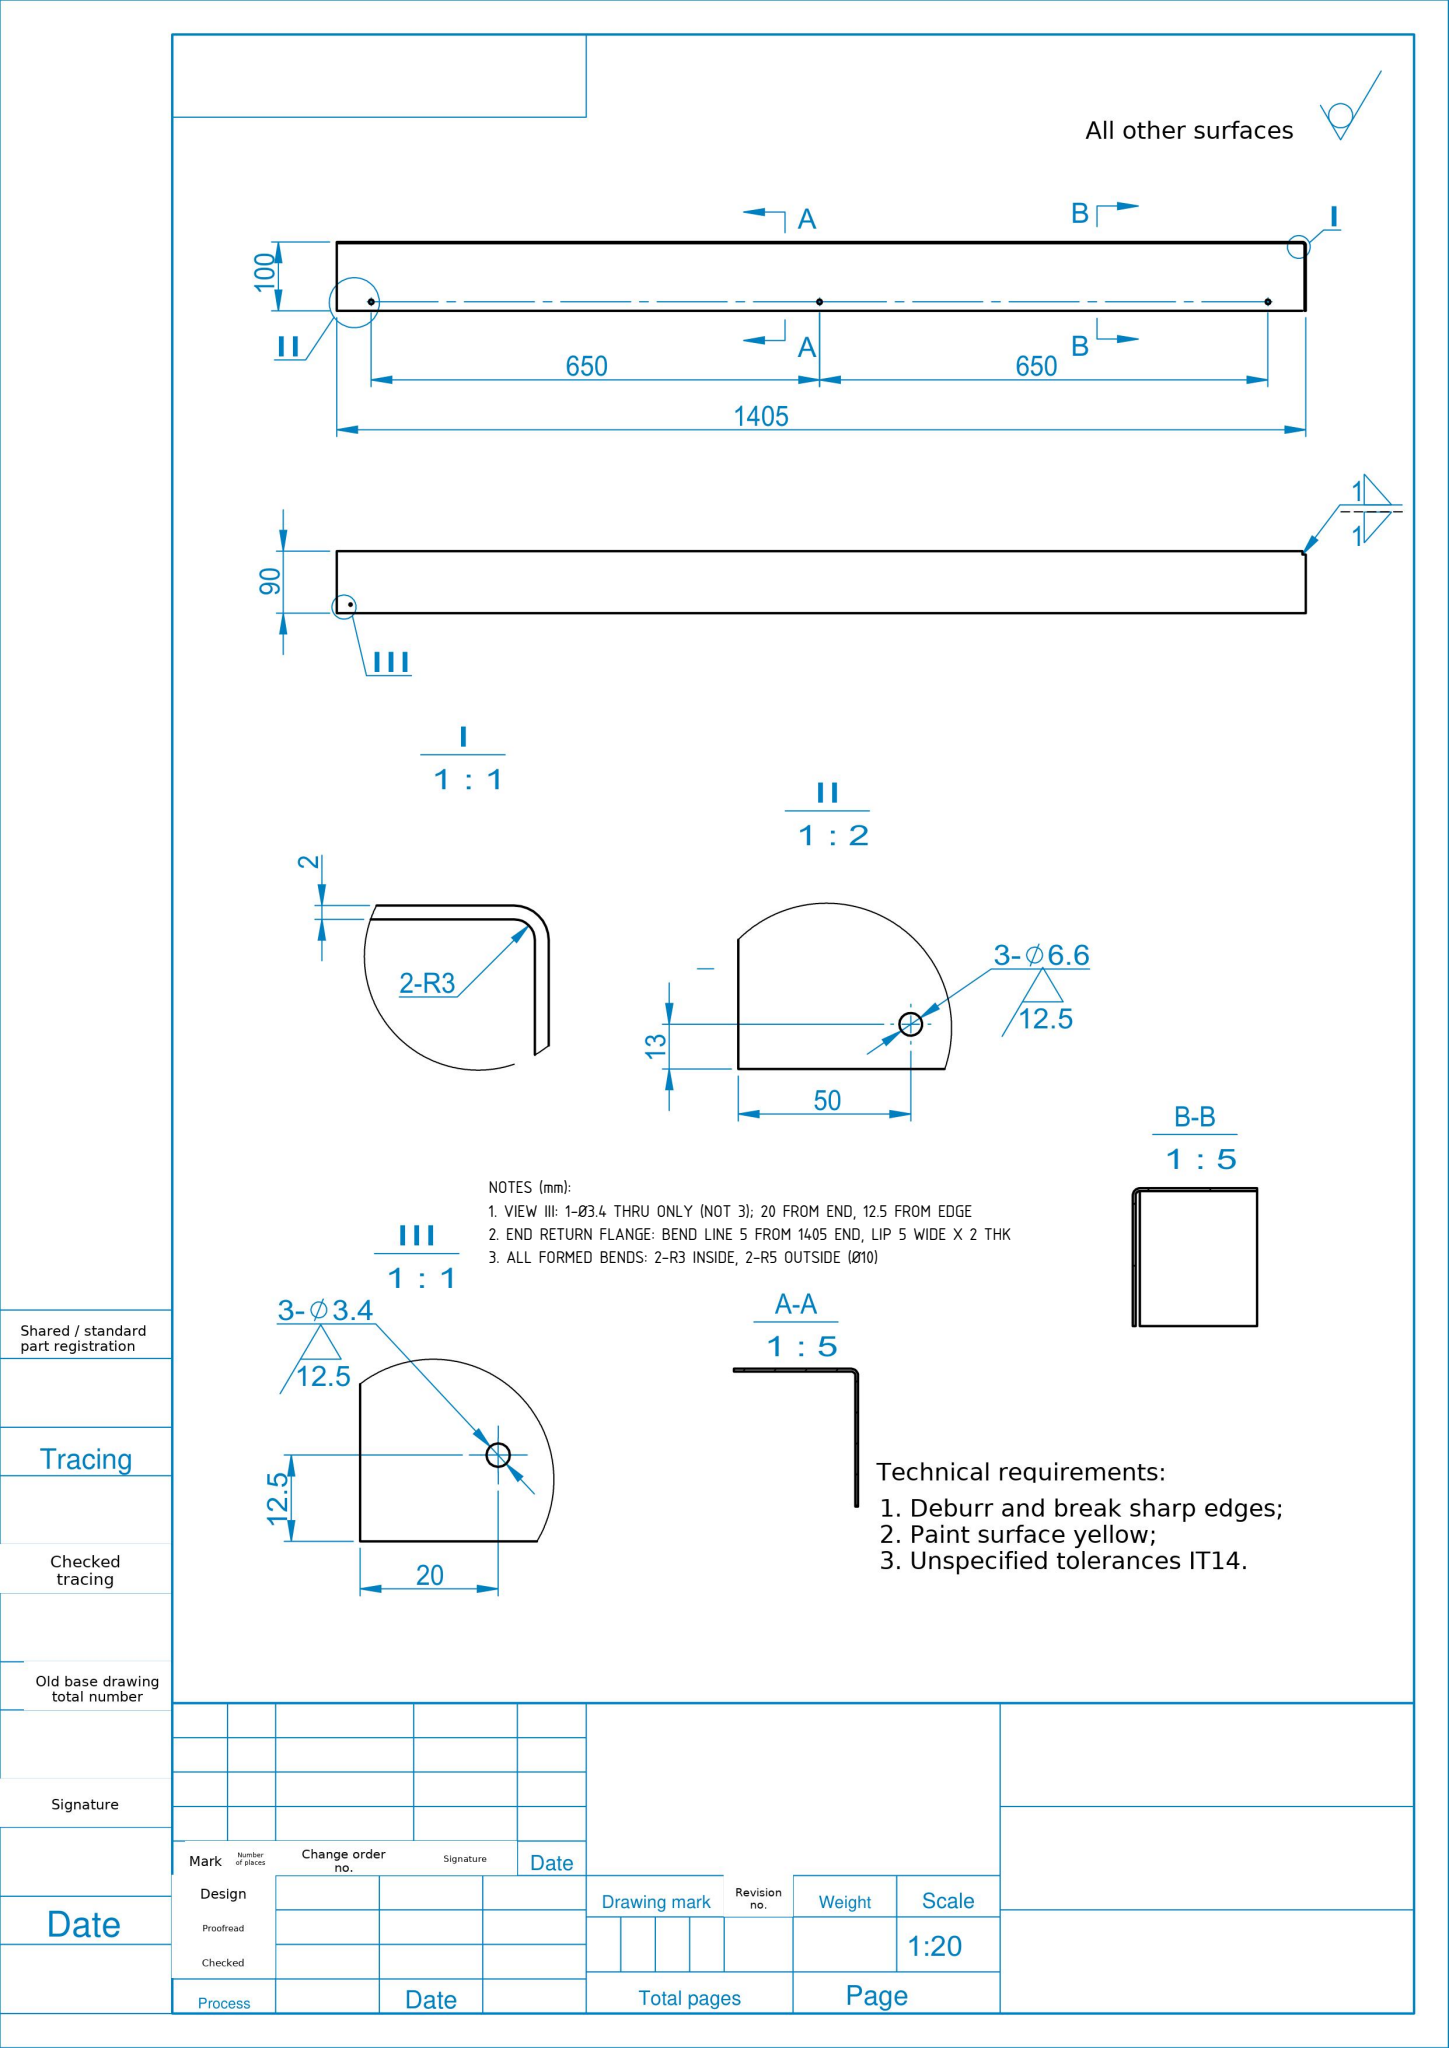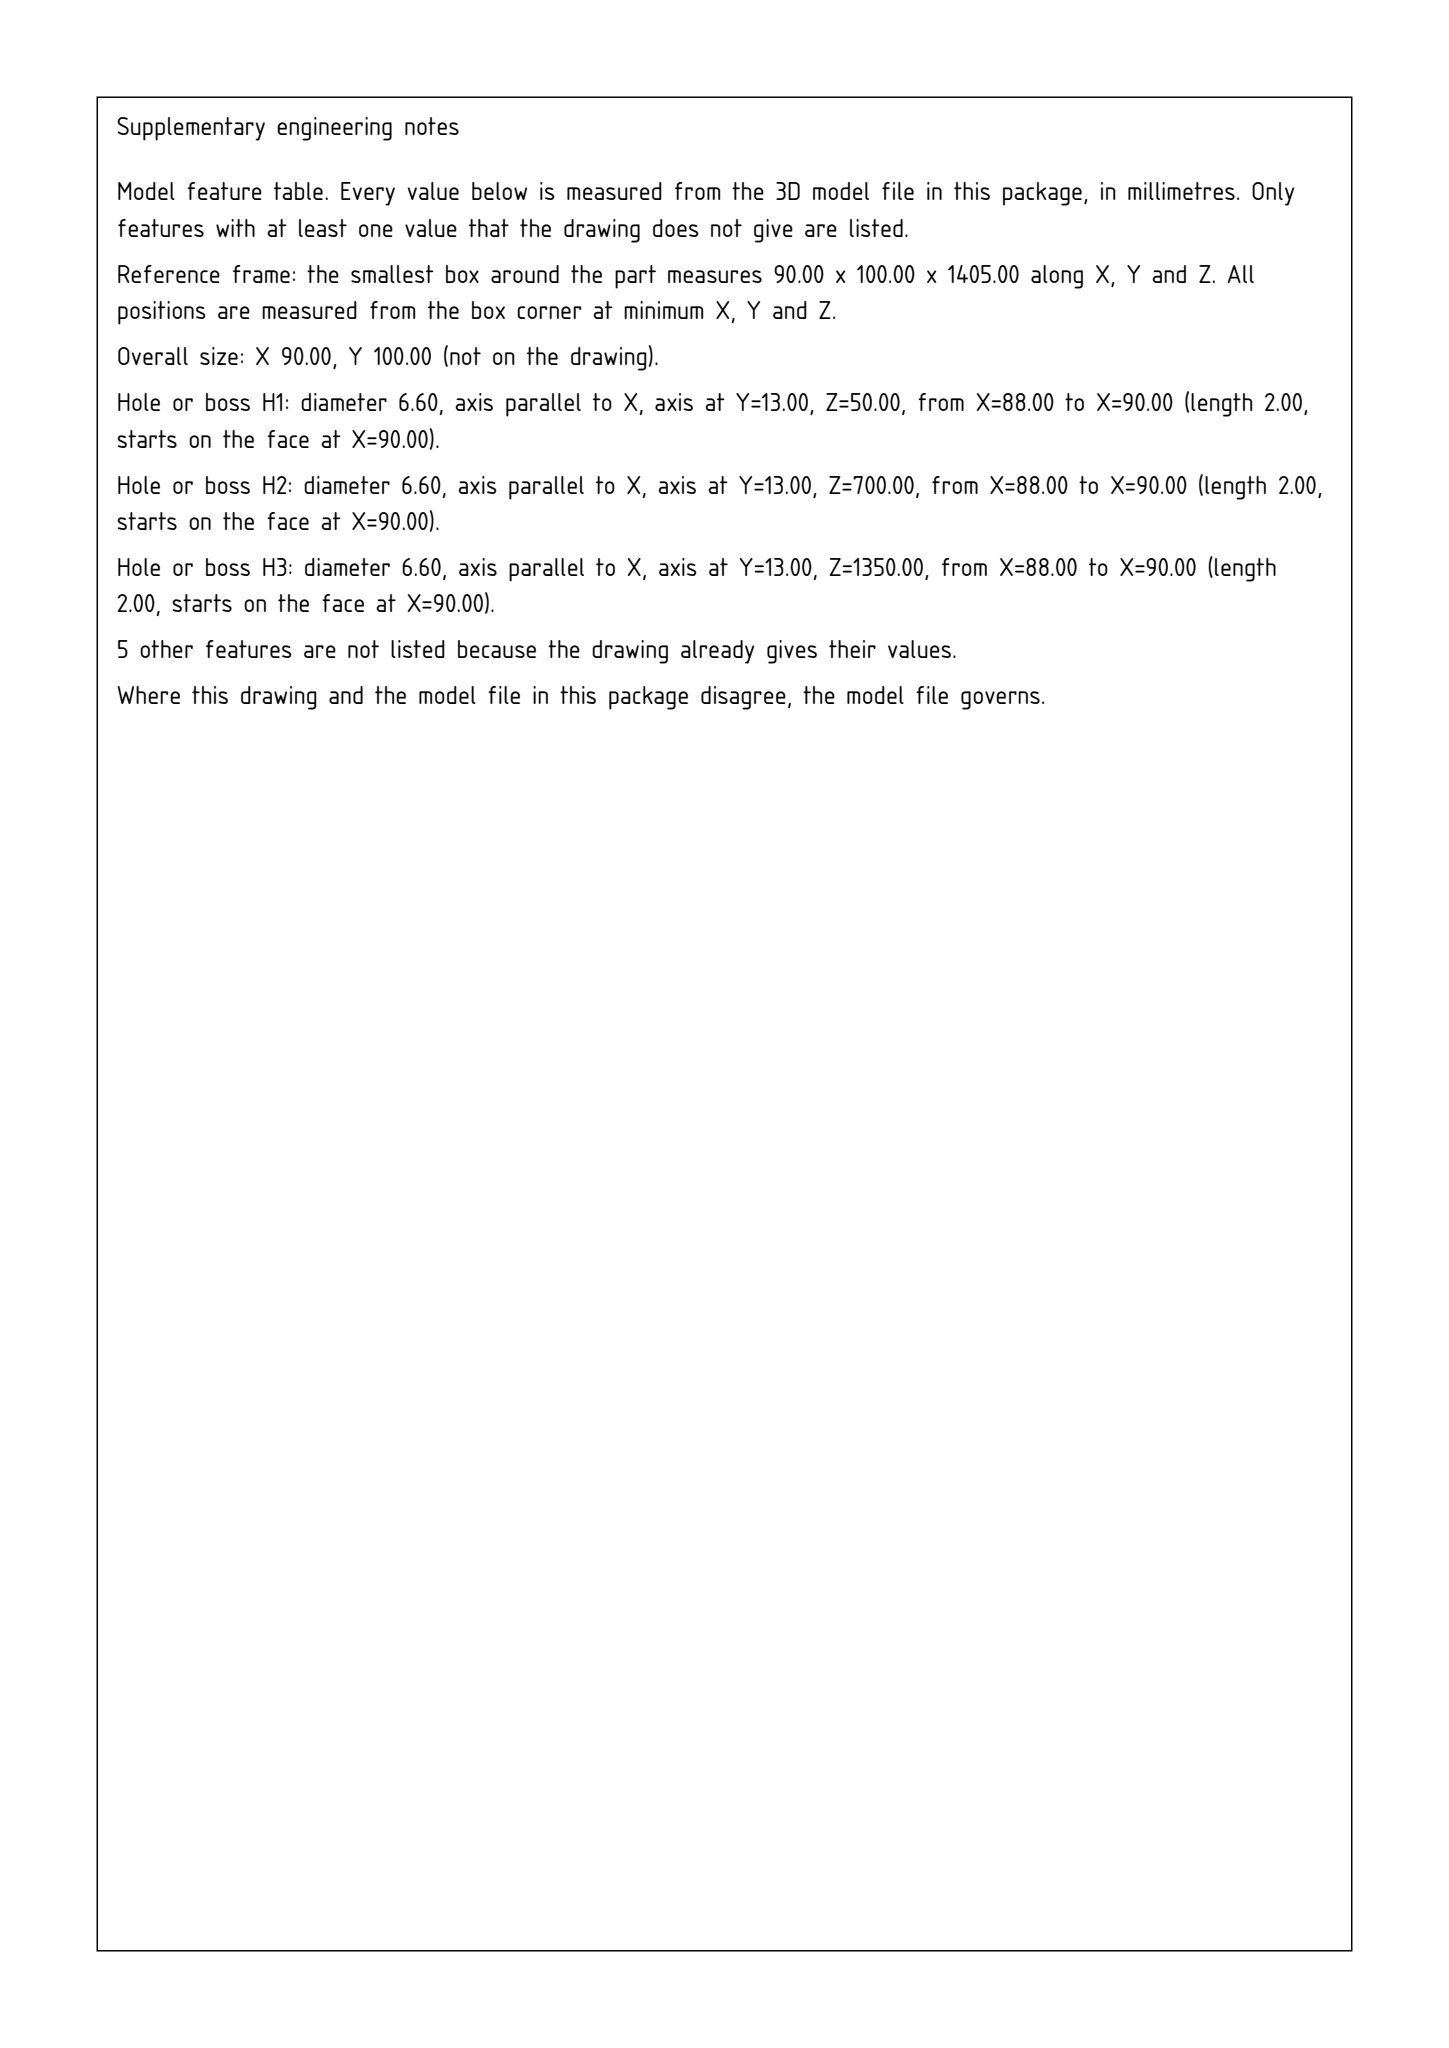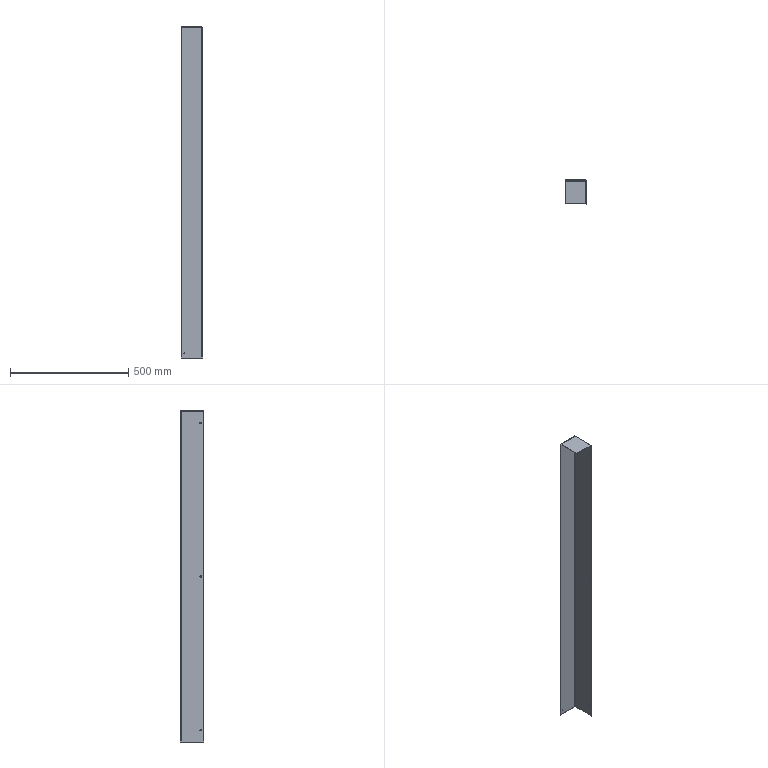Part | SolidWorks | mm | 1 solid | 30 faces | box 90 x 100 x 1405 mm | volume 538588 mm3 | plane 18 | cylinder 12 | commonest cylinder face diameters 6.6 x6 3.4 x2 10 x2 6 x2
Drawing notes:
VIEW III: 1-Ø3.4 THRU ONLY (NOT 3); 20 FROM END, 12.5 FROM EDGE | from the solid: cylinders dia 3.4, axis y, pos (x=12.5, z=20.0), len 2.0 - single location; no other Ø3.4 cylinders in model
END RETURN FLANGE: BEND LINE 5 FROM 1405 END, LIP 5 WIDE X 2 THK | from the solid: Cyl Ø6/Ø10 about x-axis at y=95, z=1400; planes z=1400/1403/1405, y=98/100
ALL FORMED BENDS: 2-R3 INSIDE, 2-R5 OUTSIDE (Ø10) | from the solid: Ø6 inner / Ø10 outer bend cylinders (x-axis at y=95,z=1400; z-axis at x=85,y=95)
STEP:
#1=CARTESIAN_POINT('',(0.,13.,-1346.7));
#2=VERTEX_POINT('',#1);
#3=CARTESIAN_POINT('',(0.,13.,-1353.3));
#4=VERTEX_POINT('',#3);
#5=CARTESIAN_POINT('',(0.,13.,-1350.));
#6=DIRECTION('',(1.,0.,-0.));
#7=DIRECTION('',(0.,-0.,-1.));
#8=AXIS2_PLACEMENT_3D('',#5,#6,#7);
#9=CIRCLE('',#8,3.3);
#10=EDGE_CURVE('',#2,#4,#9,.T.);
#11=ORIENTED_EDGE('',*,*,#10,.F.);
#12=CARTESIAN_POINT('',(2.,13.,-1346.7));
#13=VERTEX_POINT('',#12);
#14=CARTESIAN_POINT('',(2.,13.,-1346.7));
#15=DIRECTION('',(1.,0.,-0.));
#16=VECTOR('',#15,1000.);
#17=LINE('',#14,#16);
#18=EDGE_CURVE('',#2,#13,#17,.T.);
#19=ORIENTED_EDGE('',*,*,#18,.T.);
#20=CARTESIAN_POINT('',(2.,13.,-1353.3));
#21=VERTEX_POINT('',#20);
#22=CARTESIAN_POINT('',(2.,13.,-1350.));
#23=DIRECTION('',(1.,0.,-0.));
#24=DIRECTION('',(0.,-0.,-1.));
#25=AXIS2_PLACEMENT_3D('',#22,#23,#24);
#26=CIRCLE('',#25,3.3);
#27=EDGE_CURVE('',#13,#21,#26,.T.);
#28=ORIENTED_EDGE('',*,*,#27,.T.);
#29=CARTESIAN_POINT('',(2.,13.,-1353.3));
#30=DIRECTION('',(1.,0.,-0.));
#31=VECTOR('',#30,1000.);
#32=LINE('',#29,#31);
#33=EDGE_CURVE('',#4,#21,#32,.T.);
#34=ORIENTED_EDGE('',*,*,#33,.F.);
#35=EDGE_LOOP('',(#11,#19,#28,#34));
#36=FACE_OUTER_BOUND('',#35,.T.);
#37=CARTESIAN_POINT('',(2.,13.,-1350.));
#38=DIRECTION('',(1.,0.,-0.));
#39=DIRECTION('',(0.,-0.,-1.));
#40=AXIS2_PLACEMENT_3D('',#37,#38,#39);
#41=CYLINDRICAL_SURFACE('',#40,3.3);
#42=ADVANCED_FACE('',(#36),#41,.F.);
#43=CARTESIAN_POINT('',(0.,13.,-696.7));
#44=VERTEX_POINT('',#43);
#45=CARTESIAN_POINT('',(0.,13.,-703.3));
#46=VERTEX_POINT('',#45);
#47=CARTESIAN_POINT('',(0.,13.,-700.));
#48=DIRECTION('',(1.,0.,-0.));
#49=DIRECTION('',(0.,-0.,-1.));
#50=AXIS2_PLACEMENT_3D('',#47,#48,#49);
#51=CIRCLE('',#50,3.3);
#52=EDGE_CURVE('',#44,#46,#51,.T.);
#53=ORIENTED_EDGE('',*,*,#52,.F.);
#54=CARTESIAN_POINT('',(2.,13.,-696.7));
#55=VERTEX_POINT('',#54);
#56=CARTESIAN_POINT('',(2.,13.,-696.7));
#57=DIRECTION('',(1.,0.,-0.));
#58=VECTOR('',#57,1000.);
#59=LINE('',#56,#58);
#60=EDGE_CURVE('',#44,#55,#59,.T.);
#61=ORIENTED_EDGE('',*,*,#60,.T.);
#62=CARTESIAN_POINT('',(2.,13.,-703.3));
#63=VERTEX_POINT('',#62);
#64=CARTESIAN_POINT('',(2.,13.,-700.));
#65=DIRECTION('',(1.,0.,-0.));
#66=DIRECTION('',(0.,-0.,-1.));
#67=AXIS2_PLACEMENT_3D('',#64,#65,#66);
#68=CIRCLE('',#67,3.3);
#69=EDGE_CURVE('',#55,#63,#68,.T.);
#70=ORIENTED_EDGE('',*,*,#69,.T.);
#71=CARTESIAN_POINT('',(2.,13.,-703.3));
#72=DIRECTION('',(1.,0.,-0.));
#73=VECTOR('',#72,1000.);
#74=LINE('',#71,#73);
#75=EDGE_CURVE('',#46,#63,#74,.T.);
#76=ORIENTED_EDGE('',*,*,#75,.F.);
#77=EDGE_LOOP('',(#53,#61,#70,#76));
#78=FACE_OUTER_BOUND('',#77,.T.);
#79=CARTESIAN_POINT('',(2.,13.,-700.));
#80=DIRECTION('',(1.,0.,-0.));
#81=DIRECTION('',(0.,-0.,-1.));
#82=AXIS2_PLACEMENT_3D('',#79,#80,#81);
#83=CYLINDRICAL_SURFACE('',#82,3.3);
#84=ADVANCED_FACE('',(#78),#83,.F.);
#85=CARTESIAN_POINT('',(-0.,13.,-46.7));
#86=VERTEX_POINT('',#85);
#87=CARTESIAN_POINT('',(-0.,13.,-53.3));
#88=VERTEX_POINT('',#87);
#89=CARTESIAN_POINT('',(-0.,13.,-50.));
#90=DIRECTION('',(1.,0.,-0.));
#91=DIRECTION('',(0.,-0.,-1.));
#92=AXIS2_PLACEMENT_3D('',#89,#90,#91);
#93=CIRCLE('',#92,3.3);
#94=EDGE_CURVE('',#86,#88,#93,.T.);
#95=ORIENTED_EDGE('',*,*,#94,.F.);
#96=CARTESIAN_POINT('',(2.,13.,-46.7));
#97=VERTEX_POINT('',#96);
#98=CARTESIAN_POINT('',(2.,13.,-46.7));
#99=DIRECTION('',(1.,0.,-0.));
#100=VECTOR('',#99,1000.);
#101=LINE('',#98,#100);
#102=EDGE_CURVE('',#86,#97,#101,.T.);
#103=ORIENTED_EDGE('',*,*,#102,.T.);
#104=CARTESIAN_POINT('',(2.,13.,-53.3));
#105=VERTEX_POINT('',#104);
#106=CARTESIAN_POINT('',(2.,13.,-50.));
#107=DIRECTION('',(1.,0.,-0.));
#108=DIRECTION('',(0.,-0.,-1.));
#109=AXIS2_PLACEMENT_3D('',#106,#107,#108);
#110=CIRCLE('',#109,3.3);
#111=EDGE_CURVE('',#97,#105,#110,.T.);
#112=ORIENTED_EDGE('',*,*,#111,.T.);
#113=CARTESIAN_POINT('',(2.,13.,-53.3));
#114=DIRECTION('',(1.,0.,-0.));
#115=VECTOR('',#114,1000.);
#116=LINE('',#113,#115);
#117=EDGE_CURVE('',#88,#105,#116,.T.);
#118=ORIENTED_EDGE('',*,*,#117,.F.);
#119=EDGE_LOOP('',(#95,#103,#112,#118));
#120=FACE_OUTER_BOUND('',#119,.T.);
#121=CARTESIAN_POINT('',(2.,13.,-50.));
#122=DIRECTION('',(1.,0.,-0.));
#123=DIRECTION('',(0.,-0.,-1.));
#124=AXIS2_PLACEMENT_3D('',#121,#122,#123);
#125=CYLINDRICAL_SURFACE('',#124,3.3);
#126=ADVANCED_FACE('',(#120),#125,.F.);
#127=CARTESIAN_POINT('',(-75.5,100.,-1378.3));
#128=VERTEX_POINT('',#127);
#129=CARTESIAN_POINT('',(-75.5,100.,-1381.7));
#130=VERTEX_POINT('',#129);
#131=CARTESIAN_POINT('',(-75.5,100.,-1380.));
#132=DIRECTION('',(-0.,-1.,-0.));
#133=DIRECTION('',(0.,0.,-1.));
#134=AXIS2_PLACEMENT_3D('',#131,#132,#133);
#135=CIRCLE('',#134,1.7);
#136=EDGE_CURVE('',#128,#130,#135,.T.);
#137=ORIENTED_EDGE('',*,*,#136,.F.);
#138=CARTESIAN_POINT('',(-75.5,98.,-1378.3));
#139=VERTEX_POINT('',#138);
#140=CARTESIAN_POINT('',(-75.5,98.,-1378.3));
#141=DIRECTION('',(-0.,-1.,-0.));
#142=VECTOR('',#141,1000.);
#143=LINE('',#140,#142);
#144=EDGE_CURVE('',#128,#139,#143,.T.);
#145=ORIENTED_EDGE('',*,*,#144,.T.);
#146=CARTESIAN_POINT('',(-75.5,98.,-1381.7));
#147=VERTEX_POINT('',#146);
#148=CARTESIAN_POINT('',(-75.5,98.,-1380.));
#149=DIRECTION('',(-0.,-1.,-0.));
#150=DIRECTION('',(0.,0.,-1.));
#151=AXIS2_PLACEMENT_3D('',#148,#149,#150);
#152=CIRCLE('',#151,1.7);
#153=EDGE_CURVE('',#139,#147,#152,.T.);
#154=ORIENTED_EDGE('',*,*,#153,.T.);
#155=CARTESIAN_POINT('',(-75.5,98.,-1381.7));
#156=DIRECTION('',(-0.,-1.,-0.));
#157=VECTOR('',#156,1000.);
#158=LINE('',#155,#157);
#159=EDGE_CURVE('',#130,#147,#158,.T.);
#160=ORIENTED_EDGE('',*,*,#159,.F.);
#161=EDGE_LOOP('',(#137,#145,#154,#160));
#162=FACE_OUTER_BOUND('',#161,.T.);
#163=CARTESIAN_POINT('',(-75.5,98.,-1380.));
#164=DIRECTION('',(-0.,-1.,-0.));
#165=DIRECTION('',(0.,0.,-1.));
#166=AXIS2_PLACEMENT_3D('',#163,#164,#165);
#167=CYLINDRICAL_SURFACE('',#166,1.7);
#168=ADVANCED_FACE('',(#162),#167,.F.);
#169=CARTESIAN_POINT('',(-0.,95.,-1400.));
#170=VERTEX_POINT('',#169);
#171=CARTESIAN_POINT('',(2.,95.,-1400.));
#172=VERTEX_POINT('',#171);
#173=CARTESIAN_POINT('',(-0.,95.,-1400.));
#174=DIRECTION('',(1.,0.,-0.));
#175=VECTOR('',#174,1000.);
#176=LINE('',#173,#175);
#177=EDGE_CURVE('',#170,#172,#176,.T.);
#178=ORIENTED_EDGE('',*,*,#177,.F.);
#179=CARTESIAN_POINT('',(-3.,98.,-1400.));
#180=VERTEX_POINT('',#179);
#181=CARTESIAN_POINT('',(-3.,95.,-1400.));
#182=DIRECTION('',(-0.,0.,1.));
#183=DIRECTION('',(-1.,0.,0.));
#184=AXIS2_PLACEMENT_3D('',#181,#182,#183);
#185=CIRCLE('',#184,3.);
#186=EDGE_CURVE('',#170,#180,#185,.T.);
#187=ORIENTED_EDGE('',*,*,#186,.T.);
#188=CARTESIAN_POINT('',(-3.,100.,-1400.));
#189=VERTEX_POINT('',#188);
#190=CARTESIAN_POINT('',(-3.,100.,-1400.));
#191=DIRECTION('',(-0.,-1.,-0.));
#192=VECTOR('',#191,1000.);
#193=LINE('',#190,#192);
#194=EDGE_CURVE('',#189,#180,#193,.T.);
#195=ORIENTED_EDGE('',*,*,#194,.F.);
#196=CARTESIAN_POINT('',(-3.,95.,-1400.));
#197=DIRECTION('',(-0.,0.,1.));
#198=DIRECTION('',(1.,0.,0.));
#199=AXIS2_PLACEMENT_3D('',#196,#197,#198);
#200=CIRCLE('',#199,5.);
#201=EDGE_CURVE('',#172,#189,#200,.T.);
#202=ORIENTED_EDGE('',*,*,#201,.F.);
#203=EDGE_LOOP('',(#178,#187,#195,#202));
#204=FACE_OUTER_BOUND('',#203,.T.);
#205=CARTESIAN_POINT('',(-0.,95.,-1400.));
#206=DIRECTION('',(-0.,-0.,-1.));
#207=DIRECTION('',(-1.,-0.,0.));
#208=AXIS2_PLACEMENT_3D('',#205,#206,#207);
#209=PLANE('',#208);
#210=ADVANCED_FACE('',(#204),#209,.T.);
#211=CARTESIAN_POINT('',(-0.,-0.,-1400.));
#212=VERTEX_POINT('',#211);
#213=CARTESIAN_POINT('',(-0.,-0.,-1400.));
#214=DIRECTION('',(0.,1.,0.));
#215=VECTOR('',#214,1000.);
#216=LINE('',#213,#215);
#217=EDGE_CURVE('',#212,#170,#216,.T.);
#218=ORIENTED_EDGE('',*,*,#217,.T.);
#219=ORIENTED_EDGE('',*,*,#177,.T.);
#220=CARTESIAN_POINT('',(2.,-0.,-1400.));
#221=VERTEX_POINT('',#220);
#222=CARTESIAN_POINT('',(2.,-0.,-1400.));
#223=DIRECTION('',(0.,1.,0.));
#224=VECTOR('',#223,1000.);
#225=LINE('',#222,#224);
#226=EDGE_CURVE('',#221,#172,#225,.T.);
#227=ORIENTED_EDGE('',*,*,#226,.F.);
#228=CARTESIAN_POINT('',(2.,-0.,-1400.));
#229=DIRECTION('',(-1.,-0.,0.));
#230=VECTOR('',#229,1000.);
#231=LINE('',#228,#230);
#232=EDGE_CURVE('',#221,#212,#231,.T.);
#233=ORIENTED_EDGE('',*,*,#232,.T.);
#234=EDGE_LOOP('',(#218,#219,#227,#233));
#235=FACE_OUTER_BOUND('',#234,.T.);
#236=CARTESIAN_POINT('',(-3.,100.,-1400.));
#237=DIRECTION('',(-0.,-0.,-1.));
#238=DIRECTION('',(-1.,-0.,0.));
#239=AXIS2_PLACEMENT_3D('',#236,#237,#238);
#240=PLANE('',#239);
#241=ADVANCED_FACE('',(#235),#240,.T.);
#242=CARTESIAN_POINT('',(-3.,98.,0.));
#243=VERTEX_POINT('',#242);
#244=CARTESIAN_POINT('',(-3.,100.,0.));
#245=VERTEX_POINT('',#244);
#246=CARTESIAN_POINT('',(-3.,98.,0.));
#247=DIRECTION('',(0.,1.,0.));
#248=VECTOR('',#247,1000.);
#249=LINE('',#246,#248);
#250=EDGE_CURVE('',#243,#245,#249,.T.);
#251=ORIENTED_EDGE('',*,*,#250,.F.);
#252=CARTESIAN_POINT('',(0.,95.,0.));
#253=VERTEX_POINT('',#252);
#254=CARTESIAN_POINT('',(-3.,95.,0.));
#255=DIRECTION('',(-0.,0.,1.));
#256=DIRECTION('',(-1.,0.,0.));
#257=AXIS2_PLACEMENT_3D('',#254,#255,#256);
#258=CIRCLE('',#257,3.);
#259=EDGE_CURVE('',#253,#243,#258,.T.);
#260=ORIENTED_EDGE('',*,*,#259,.F.);
#261=CARTESIAN_POINT('',(2.,95.,0.));
#262=VERTEX_POINT('',#261);
#263=CARTESIAN_POINT('',(2.,95.,0.));
#264=DIRECTION('',(-1.,-0.,0.));
#265=VECTOR('',#264,1000.);
#266=LINE('',#263,#265);
#267=EDGE_CURVE('',#262,#253,#266,.T.);
#268=ORIENTED_EDGE('',*,*,#267,.F.);
#269=CARTESIAN_POINT('',(-3.,95.,0.));
#270=DIRECTION('',(-0.,0.,1.));
#271=DIRECTION('',(1.,0.,-0.));
#272=AXIS2_PLACEMENT_3D('',#269,#270,#271);
#273=CIRCLE('',#272,5.);
#274=EDGE_CURVE('',#262,#245,#273,.T.);
#275=ORIENTED_EDGE('',*,*,#274,.T.);
#276=EDGE_LOOP('',(#251,#260,#268,#275));
#277=FACE_OUTER_BOUND('',#276,.T.);
#278=CARTESIAN_POINT('',(-3.,98.,0.));
#279=DIRECTION('',(0.,0.,1.));
#280=DIRECTION('',(1.,0.,-0.));
#281=AXIS2_PLACEMENT_3D('',#278,#279,#280);
#282=PLANE('',#281);
#283=ADVANCED_FACE('',(#277),#282,.T.);
#284=CARTESIAN_POINT('',(-75.5,100.,-1380.));
#285=DIRECTION('',(-0.,-1.,-0.));
#286=DIRECTION('',(0.,0.,-1.));
#287=AXIS2_PLACEMENT_3D('',#284,#285,#286);
#288=CIRCLE('',#287,1.7);
#289=EDGE_CURVE('',#130,#128,#288,.T.);
#290=ORIENTED_EDGE('',*,*,#289,.T.);
#291=ORIENTED_EDGE('',*,*,#136,.T.);
#292=EDGE_LOOP('',(#290,#291));
#293=FACE_BOUND('',#292,.T.);
#294=CARTESIAN_POINT('',(-88.,100.,0.));
#295=VERTEX_POINT('',#294);
#296=CARTESIAN_POINT('',(-0.,100.,0.));
#297=DIRECTION('',(-1.,-0.,0.));
#298=VECTOR('',#297,1000.);
#299=LINE('',#296,#298);
#300=EDGE_CURVE('',#245,#295,#299,.T.);
#301=ORIENTED_EDGE('',*,*,#300,.F.);
#302=CARTESIAN_POINT('',(-3.,100.,-1400.));
#303=DIRECTION('',(-0.,0.,1.));
#304=VECTOR('',#303,1000.);
#305=LINE('',#302,#304);
#306=EDGE_CURVE('',#189,#245,#305,.T.);
#307=ORIENTED_EDGE('',*,*,#306,.F.);
#308=CARTESIAN_POINT('',(-88.,100.,-1400.));
#309=VERTEX_POINT('',#308);
#310=CARTESIAN_POINT('',(0.,100.,-1400.));
#311=DIRECTION('',(-1.,-0.,0.));
#312=VECTOR('',#311,1000.);
#313=LINE('',#310,#312);
#314=EDGE_CURVE('',#189,#309,#313,.T.);
#315=ORIENTED_EDGE('',*,*,#314,.T.);
#316=CARTESIAN_POINT('',(-88.,100.,-1400.));
#317=DIRECTION('',(-0.,0.,1.));
#318=VECTOR('',#317,1000.);
#319=LINE('',#316,#318);
#320=EDGE_CURVE('',#309,#295,#319,.T.);
#321=ORIENTED_EDGE('',*,*,#320,.T.);
#322=EDGE_LOOP('',(#301,#307,#315,#321));
#323=FACE_OUTER_BOUND('',#322,.T.);
#324=CARTESIAN_POINT('',(0.,100.,-1400.));
#325=DIRECTION('',(0.,1.,-0.));
#326=DIRECTION('',(-0.,0.,1.));
#327=AXIS2_PLACEMENT_3D('',#324,#325,#326);
#328=PLANE('',#327);
#329=ADVANCED_FACE('',(#293,#323),#328,.T.);
#330=ORIENTED_EDGE('',*,*,#274,.F.);
#331=CARTESIAN_POINT('',(2.,95.,-1400.));
#332=DIRECTION('',(-0.,0.,1.));
#333=VECTOR('',#332,1000.);
#334=LINE('',#331,#333);
#335=EDGE_CURVE('',#172,#262,#334,.T.);
#336=ORIENTED_EDGE('',*,*,#335,.F.);
#337=ORIENTED_EDGE('',*,*,#201,.T.);
#338=ORIENTED_EDGE('',*,*,#306,.T.);
#339=EDGE_LOOP('',(#330,#336,#337,#338));
#340=FACE_OUTER_BOUND('',#339,.T.);
#341=CARTESIAN_POINT('',(-3.,95.,-1400.));
#342=DIRECTION('',(-0.,0.,1.));
#343=DIRECTION('',(1.,0.,0.));
#344=AXIS2_PLACEMENT_3D('',#341,#342,#343);
#345=CYLINDRICAL_SURFACE('',#344,5.);
#346=ADVANCED_FACE('',(#340),#345,.T.);
#347=CARTESIAN_POINT('',(2.,13.,-1350.));
#348=DIRECTION('',(1.,0.,-0.));
#349=DIRECTION('',(0.,-0.,-1.));
#350=AXIS2_PLACEMENT_3D('',#347,#348,#349);
#351=CIRCLE('',#350,3.3);
#352=EDGE_CURVE('',#21,#13,#351,.T.);
#353=ORIENTED_EDGE('',*,*,#352,.F.);
#354=ORIENTED_EDGE('',*,*,#27,.F.);
#355=EDGE_LOOP('',(#353,#354));
#356=FACE_BOUND('',#355,.T.);
#357=CARTESIAN_POINT('',(2.,13.,-700.));
#358=DIRECTION('',(1.,0.,-0.));
#359=DIRECTION('',(0.,-0.,-1.));
#360=AXIS2_PLACEMENT_3D('',#357,#358,#359);
#361=CIRCLE('',#360,3.3);
#362=EDGE_CURVE('',#63,#55,#361,.T.);
#363=ORIENTED_EDGE('',*,*,#362,.F.);
#364=ORIENTED_EDGE('',*,*,#69,.F.);
#365=EDGE_LOOP('',(#363,#364));
#366=FACE_BOUND('',#365,.T.);
#367=CARTESIAN_POINT('',(2.,13.,-50.));
#368=DIRECTION('',(1.,0.,-0.));
#369=DIRECTION('',(0.,-0.,-1.));
#370=AXIS2_PLACEMENT_3D('',#367,#368,#369);
#371=CIRCLE('',#370,3.3);
#372=EDGE_CURVE('',#105,#97,#371,.T.);
#373=ORIENTED_EDGE('',*,*,#372,.F.);
#374=ORIENTED_EDGE('',*,*,#111,.F.);
#375=EDGE_LOOP('',(#373,#374));
#376=FACE_BOUND('',#375,.T.);
#377=CARTESIAN_POINT('',(2.,0.,0.));
#378=VERTEX_POINT('',#377);
#379=CARTESIAN_POINT('',(2.,0.,0.));
#380=DIRECTION('',(0.,1.,0.));
#381=VECTOR('',#380,1000.);
#382=LINE('',#379,#381);
#383=EDGE_CURVE('',#378,#262,#382,.T.);
#384=ORIENTED_EDGE('',*,*,#383,.F.);
#385=CARTESIAN_POINT('',(2.,-0.,-1400.));
#386=DIRECTION('',(-0.,0.,1.));
#387=VECTOR('',#386,1000.);
#388=LINE('',#385,#387);
#389=EDGE_CURVE('',#221,#378,#388,.T.);
#390=ORIENTED_EDGE('',*,*,#389,.F.);
#391=ORIENTED_EDGE('',*,*,#226,.T.);
#392=ORIENTED_EDGE('',*,*,#335,.T.);
#393=EDGE_LOOP('',(#384,#390,#391,#392));
#394=FACE_OUTER_BOUND('',#393,.T.);
#395=CARTESIAN_POINT('',(2.,-0.,-1400.));
#396=DIRECTION('',(1.,0.,0.));
#397=DIRECTION('',(0.,-0.,-1.));
#398=AXIS2_PLACEMENT_3D('',#395,#396,#397);
#399=PLANE('',#398);
#400=ADVANCED_FACE('',(#356,#366,#376,#394),#399,.T.);
#401=CARTESIAN_POINT('',(0.,0.,0.));
#402=VERTEX_POINT('',#401);
#403=CARTESIAN_POINT('',(2.,0.,0.));
#404=DIRECTION('',(-1.,-0.,0.));
#405=VECTOR('',#404,1000.);
#406=LINE('',#403,#405);
#407=EDGE_CURVE('',#378,#402,#406,.T.);
#408=ORIENTED_EDGE('',*,*,#407,.T.);
#409=CARTESIAN_POINT('',(-0.,-0.,-1400.));
#410=DIRECTION('',(-0.,0.,1.));
#411=VECTOR('',#410,1000.);
#412=LINE('',#409,#411);
#413=EDGE_CURVE('',#212,#402,#412,.T.);
#414=ORIENTED_EDGE('',*,*,#413,.F.);
#415=ORIENTED_EDGE('',*,*,#232,.F.);
#416=ORIENTED_EDGE('',*,*,#389,.T.);
#417=EDGE_LOOP('',(#408,#414,#415,#416));
#418=FACE_OUTER_BOUND('',#417,.T.);
#419=CARTESIAN_POINT('',(2.,-0.,-1400.));
#420=DIRECTION('',(0.,1.,-0.));
#421=DIRECTION('',(-0.,0.,1.));
#422=AXIS2_PLACEMENT_3D('',#419,#420,#421);
#423=PLANE('',#422);
#424=ADVANCED_FACE('',(#418),#423,.F.);
#425=CARTESIAN_POINT('',(0.,13.,-1350.));
#426=DIRECTION('',(1.,0.,-0.));
#427=DIRECTION('',(0.,-0.,-1.));
#428=AXIS2_PLACEMENT_3D('',#425,#426,#427);
#429=CIRCLE('',#428,3.3);
#430=EDGE_CURVE('',#4,#2,#429,.T.);
#431=ORIENTED_EDGE('',*,*,#430,.T.);
#432=ORIENTED_EDGE('',*,*,#10,.T.);
#433=EDGE_LOOP('',(#431,#432));
#434=FACE_BOUND('',#433,.T.);
#435=CARTESIAN_POINT('',(0.,13.,-700.));
#436=DIRECTION('',(1.,0.,-0.));
#437=DIRECTION('',(0.,-0.,-1.));
#438=AXIS2_PLACEMENT_3D('',#435,#436,#437);
#439=CIRCLE('',#438,3.3);
#440=EDGE_CURVE('',#46,#44,#439,.T.);
#441=ORIENTED_EDGE('',*,*,#440,.T.);
#442=ORIENTED_EDGE('',*,*,#52,.T.);
#443=EDGE_LOOP('',(#441,#442));
#444=FACE_BOUND('',#443,.T.);
#445=CARTESIAN_POINT('',(-0.,13.,-50.));
#446=DIRECTION('',(1.,0.,-0.));
#447=DIRECTION('',(0.,-0.,-1.));
#448=AXIS2_PLACEMENT_3D('',#445,#446,#447);
#449=CIRCLE('',#448,3.3);
#450=EDGE_CURVE('',#88,#86,#449,.T.);
#451=ORIENTED_EDGE('',*,*,#450,.T.);
#452=ORIENTED_EDGE('',*,*,#94,.T.);
#453=EDGE_LOOP('',(#451,#452));
#454=FACE_BOUND('',#453,.T.);
#455=CARTESIAN_POINT('',(0.,0.,0.));
#456=DIRECTION('',(0.,1.,0.));
#457=VECTOR('',#456,1000.);
#458=LINE('',#455,#457);
#459=EDGE_CURVE('',#402,#253,#458,.T.);
#460=ORIENTED_EDGE('',*,*,#459,.T.);
#461=CARTESIAN_POINT('',(-0.,95.,-1400.));
#462=DIRECTION('',(-0.,0.,1.));
#463=VECTOR('',#462,1000.);
#464=LINE('',#461,#463);
#465=EDGE_CURVE('',#170,#253,#464,.T.);
#466=ORIENTED_EDGE('',*,*,#465,.F.);
#467=ORIENTED_EDGE('',*,*,#217,.F.);
#468=ORIENTED_EDGE('',*,*,#413,.T.);
#469=EDGE_LOOP('',(#460,#466,#467,#468));
#470=FACE_OUTER_BOUND('',#469,.T.);
#471=CARTESIAN_POINT('',(-0.,-0.,-1400.));
#472=DIRECTION('',(1.,0.,0.));
#473=DIRECTION('',(0.,-0.,-1.));
#474=AXIS2_PLACEMENT_3D('',#471,#472,#473);
#475=PLANE('',#474);
#476=ADVANCED_FACE('',(#434,#444,#454,#470),#475,.F.);
#477=ORIENTED_EDGE('',*,*,#259,.T.);
#478=CARTESIAN_POINT('',(-3.,98.,-1400.));
#479=DIRECTION('',(-0.,0.,1.));
#480=VECTOR('',#479,1000.);
#481=LINE('',#478,#480);
#482=EDGE_CURVE('',#180,#243,#481,.T.);
#483=ORIENTED_EDGE('',*,*,#482,.F.);
#484=ORIENTED_EDGE('',*,*,#186,.F.);
#485=ORIENTED_EDGE('',*,*,#465,.T.);
#486=EDGE_LOOP('',(#477,#483,#484,#485));
#487=FACE_OUTER_BOUND('',#486,.T.);
#488=CARTESIAN_POINT('',(-3.,95.,-1400.));
#489=DIRECTION('',(-0.,0.,1.));
#490=DIRECTION('',(1.,0.,0.));
#491=AXIS2_PLACEMENT_3D('',#488,#489,#490);
#492=CYLINDRICAL_SURFACE('',#491,3.);
#493=ADVANCED_FACE('',(#487),#492,.F.);
#494=CARTESIAN_POINT('',(-75.5,98.,-1380.));
#495=DIRECTION('',(-0.,-1.,-0.));
#496=DIRECTION('',(0.,0.,-1.));
#497=AXIS2_PLACEMENT_3D('',#494,#495,#496);
#498=CIRCLE('',#497,1.7);
#499=EDGE_CURVE('',#147,#139,#498,.T.);
#500=ORIENTED_EDGE('',*,*,#499,.F.);
#501=ORIENTED_EDGE('',*,*,#153,.F.);
#502=EDGE_LOOP('',(#500,#501));
#503=FACE_BOUND('',#502,.T.);
#504=CARTESIAN_POINT('',(-88.,98.,0.));
#505=VERTEX_POINT('',#504);
#506=CARTESIAN_POINT('',(0.,98.,0.));
#507=DIRECTION('',(-1.,-0.,0.));
#508=VECTOR('',#507,1000.);
#509=LINE('',#506,#508);
#510=EDGE_CURVE('',#243,#505,#509,.T.);
#511=ORIENTED_EDGE('',*,*,#510,.T.);
#512=CARTESIAN_POINT('',(-88.,98.,-1400.));
#513=VERTEX_POINT('',#512);
#514=CARTESIAN_POINT('',(-88.,98.,-1400.));
#515=DIRECTION('',(-0.,0.,1.));
#516=VECTOR('',#515,1000.);
#517=LINE('',#514,#516);
#518=EDGE_CURVE('',#513,#505,#517,.T.);
#519=ORIENTED_EDGE('',*,*,#518,.F.);
#520=CARTESIAN_POINT('',(0.,98.,-1400.));
#521=DIRECTION('',(-1.,-0.,0.));
#522=VECTOR('',#521,1000.);
#523=LINE('',#520,#522);
#524=EDGE_CURVE('',#180,#513,#523,.T.);
#525=ORIENTED_EDGE('',*,*,#524,.F.);
#526=ORIENTED_EDGE('',*,*,#482,.T.);
#527=EDGE_LOOP('',(#511,#519,#525,#526));
#528=FACE_OUTER_BOUND('',#527,.T.);
#529=CARTESIAN_POINT('',(0.,98.,-1400.));
#530=DIRECTION('',(0.,1.,-0.));
#531=DIRECTION('',(-0.,0.,1.));
#532=AXIS2_PLACEMENT_3D('',#529,#530,#531);
#533=PLANE('',#532);
#534=ADVANCED_FACE('',(#503,#528),#533,.F.);
#535=CARTESIAN_POINT('',(-88.,98.,0.));
#536=DIRECTION('',(0.,1.,0.));
#537=VECTOR('',#536,1000.);
#538=LINE('',#535,#537);
#539=EDGE_CURVE('',#505,#295,#538,.T.);
#540=ORIENTED_EDGE('',*,*,#539,.T.);
#541=ORIENTED_EDGE('',*,*,#320,.F.);
#542=CARTESIAN_POINT('',(-88.,98.,-1400.));
#543=DIRECTION('',(0.,1.,0.));
#544=VECTOR('',#543,1000.);
#545=LINE('',#542,#544);
#546=EDGE_CURVE('',#513,#309,#545,.T.);
#547=ORIENTED_EDGE('',*,*,#546,.F.);
#548=ORIENTED_EDGE('',*,*,#518,.T.);
#549=EDGE_LOOP('',(#540,#541,#547,#548));
#550=FACE_OUTER_BOUND('',#549,.T.);
#551=CARTESIAN_POINT('',(-88.,98.,-1400.));
#552=DIRECTION('',(1.,0.,0.));
#553=DIRECTION('',(0.,-0.,-1.));
#554=AXIS2_PLACEMENT_3D('',#551,#552,#553);
#555=PLANE('',#554);
#556=ADVANCED_FACE('',(#550),#555,.F.);
#557=ORIENTED_EDGE('',*,*,#314,.F.);
#558=ORIENTED_EDGE('',*,*,#194,.T.);
#559=ORIENTED_EDGE('',*,*,#524,.T.);
#560=ORIENTED_EDGE('',*,*,#546,.T.);
#561=EDGE_LOOP('',(#557,#558,#559,#560));
#562=FACE_OUTER_BOUND('',#561,.T.);
#563=CARTESIAN_POINT('',(-3.,95.,-1400.));
#564=DIRECTION('',(-0.,-0.,-1.));
#565=DIRECTION('',(-1.,-0.,0.));
#566=AXIS2_PLACEMENT_3D('',#563,#564,#565);
#567=PLANE('',#566);
#568=ADVANCED_FACE('',(#562),#567,.T.);
#569=ORIENTED_EDGE('',*,*,#383,.T.);
#570=ORIENTED_EDGE('',*,*,#267,.T.);
#571=ORIENTED_EDGE('',*,*,#459,.F.);
#572=ORIENTED_EDGE('',*,*,#407,.F.);
#573=EDGE_LOOP('',(#569,#570,#571,#572));
#574=FACE_OUTER_BOUND('',#573,.T.);
#575=CARTESIAN_POINT('',(-3.,95.,0.));
#576=DIRECTION('',(-0.,-0.,-1.));
#577=DIRECTION('',(-1.,-0.,0.));
#578=AXIS2_PLACEMENT_3D('',#575,#576,#577);
#579=PLANE('',#578);
#580=ADVANCED_FACE('',(#574),#579,.F.);
#581=CARTESIAN_POINT('',(-3.,95.,3.));
#582=VERTEX_POINT('',#581);
#583=CARTESIAN_POINT('',(-3.,95.,5.));
#584=VERTEX_POINT('',#583);
#585=CARTESIAN_POINT('',(-3.,95.,5.));
#586=DIRECTION('',(-0.,0.,1.));
#587=VECTOR('',#586,1000.);
#588=LINE('',#585,#587);
#589=EDGE_CURVE('',#582,#584,#588,.T.);
#590=ORIENTED_EDGE('',*,*,#589,.F.);
#591=CARTESIAN_POINT('',(-3.,95.,0.));
#592=DIRECTION('',(1.,0.,0.));
#593=DIRECTION('',(-0.,0.,1.));
#594=AXIS2_PLACEMENT_3D('',#591,#592,#593);
#595=CIRCLE('',#594,3.);
#596=EDGE_CURVE('',#243,#582,#595,.T.);
#597=ORIENTED_EDGE('',*,*,#596,.F.);
#598=ORIENTED_EDGE('',*,*,#250,.T.);
#599=CARTESIAN_POINT('',(-3.,95.,0.));
#600=DIRECTION('',(1.,0.,0.));
#601=DIRECTION('',(-0.,0.,1.));
#602=AXIS2_PLACEMENT_3D('',#599,#600,#601);
#603=CIRCLE('',#602,5.);
#604=EDGE_CURVE('',#245,#584,#603,.T.);
#605=ORIENTED_EDGE('',*,*,#604,.T.);
#606=EDGE_LOOP('',(#590,#597,#598,#605));
#607=FACE_OUTER_BOUND('',#606,.T.);
#608=CARTESIAN_POINT('',(-3.,95.,0.));
#609=DIRECTION('',(1.,0.,0.));
#610=DIRECTION('',(0.,-0.,-1.));
#611=AXIS2_PLACEMENT_3D('',#608,#609,#610);
#612=PLANE('',#611);
#613=ADVANCED_FACE('',(#607),#612,.T.);
#614=CARTESIAN_POINT('',(-88.,95.,3.));
#615=VERTEX_POINT('',#614);
#616=CARTESIAN_POINT('',(-88.,95.,0.));
#617=DIRECTION('',(-1.,-0.,-0.));
#618=DIRECTION('',(0.,0.,1.));
#619=AXIS2_PLACEMENT_3D('',#616,#617,#618);
#620=CIRCLE('',#619,3.);
#621=EDGE_CURVE('',#615,#505,#620,.T.);
#622=ORIENTED_EDGE('',*,*,#621,.F.);
#623=CARTESIAN_POINT('',(-88.,95.,5.));
#624=VERTEX_POINT('',#623);
#625=CARTESIAN_POINT('',(-88.,95.,3.));
#626=DIRECTION('',(-0.,0.,1.));
#627=VECTOR('',#626,1000.);
#628=LINE('',#625,#627);
#629=EDGE_CURVE('',#615,#624,#628,.T.);
#630=ORIENTED_EDGE('',*,*,#629,.T.);
#631=CARTESIAN_POINT('',(-88.,95.,0.));
#632=DIRECTION('',(-1.,-0.,-0.));
#633=DIRECTION('',(0.,0.,1.));
#634=AXIS2_PLACEMENT_3D('',#631,#632,#633);
#635=CIRCLE('',#634,5.);
#636=EDGE_CURVE('',#624,#295,#635,.T.);
#637=ORIENTED_EDGE('',*,*,#636,.T.);
#638=ORIENTED_EDGE('',*,*,#539,.F.);
#639=EDGE_LOOP('',(#622,#630,#637,#638));
#640=FACE_OUTER_BOUND('',#639,.T.);
#641=CARTESIAN_POINT('',(-88.,95.,0.));
#642=DIRECTION('',(1.,0.,0.));
#643=DIRECTION('',(0.,-0.,-1.));
#644=AXIS2_PLACEMENT_3D('',#641,#642,#643);
#645=PLANE('',#644);
#646=ADVANCED_FACE('',(#640),#645,.F.);
#647=ORIENTED_EDGE('',*,*,#300,.T.);
#648=ORIENTED_EDGE('',*,*,#636,.F.);
#649=CARTESIAN_POINT('',(-3.,95.,5.));
#650=DIRECTION('',(1.,0.,-0.));
#651=VECTOR('',#650,1000.);
#652=LINE('',#649,#651);
#653=EDGE_CURVE('',#624,#584,#652,.T.);
#654=ORIENTED_EDGE('',*,*,#653,.T.);
#655=ORIENTED_EDGE('',*,*,#604,.F.);
#656=EDGE_LOOP('',(#647,#648,#654,#655));
#657=FACE_OUTER_BOUND('',#656,.T.);
#658=CARTESIAN_POINT('',(-88.,95.,0.));
#659=DIRECTION('',(-1.,-0.,-0.));
#660=DIRECTION('',(0.,0.,1.));
#661=AXIS2_PLACEMENT_3D('',#658,#659,#660);
#662=CYLINDRICAL_SURFACE('',#661,5.);
#663=ADVANCED_FACE('',(#657),#662,.T.);
#664=ORIENTED_EDGE('',*,*,#510,.F.);
#665=ORIENTED_EDGE('',*,*,#596,.T.);
#666=CARTESIAN_POINT('',(-3.,95.,3.));
#667=DIRECTION('',(-1.,-0.,0.));
#668=VECTOR('',#667,1000.);
#669=LINE('',#666,#668);
#670=EDGE_CURVE('',#582,#615,#669,.T.);
#671=ORIENTED_EDGE('',*,*,#670,.T.);
#672=ORIENTED_EDGE('',*,*,#621,.T.);
#673=EDGE_LOOP('',(#664,#665,#671,#672));
#674=FACE_OUTER_BOUND('',#673,.T.);
#675=CARTESIAN_POINT('',(-88.,95.,0.));
#676=DIRECTION('',(-1.,-0.,-0.));
#677=DIRECTION('',(0.,0.,1.));
#678=AXIS2_PLACEMENT_3D('',#675,#676,#677);
#679=CYLINDRICAL_SURFACE('',#678,3.);
#680=ADVANCED_FACE('',(#674),#679,.F.);
#681=ORIENTED_EDGE('',*,*,#629,.F.);
#682=CARTESIAN_POINT('',(-88.,0.,3.));
#683=VERTEX_POINT('',#682);
#684=CARTESIAN_POINT('',(-88.,0.,3.));
#685=DIRECTION('',(-0.,-1.,0.));
#686=VECTOR('',#685,1000.);
#687=LINE('',#684,#686);
#688=EDGE_CURVE('',#615,#683,#687,.T.);
#689=ORIENTED_EDGE('',*,*,#688,.T.);
#690=CARTESIAN_POINT('',(-88.,0.,5.));
#691=VERTEX_POINT('',#690);
#692=CARTESIAN_POINT('',(-88.,0.,5.));
#693=DIRECTION('',(0.,-0.,-1.));
#694=VECTOR('',#693,1000.);
#695=LINE('',#692,#694);
#696=EDGE_CURVE('',#691,#683,#695,.T.);
#697=ORIENTED_EDGE('',*,*,#696,.F.);
#698=CARTESIAN_POINT('',(-88.,0.,5.));
#699=DIRECTION('',(-0.,-1.,0.));
#700=VECTOR('',#699,1000.);
#701=LINE('',#698,#700);
#702=EDGE_CURVE('',#624,#691,#701,.T.);
#703=ORIENTED_EDGE('',*,*,#702,.F.);
#704=EDGE_LOOP('',(#681,#689,#697,#703));
#705=FACE_OUTER_BOUND('',#704,.T.);
#706=CARTESIAN_POINT('',(-88.,0.,5.));
#707=DIRECTION('',(1.,0.,0.));
#708=DIRECTION('',(0.,-0.,-1.));
#709=AXIS2_PLACEMENT_3D('',#706,#707,#708);
#710=PLANE('',#709);
#711=ADVANCED_FACE('',(#705),#710,.F.);
#712=ORIENTED_EDGE('',*,*,#589,.T.);
#713=CARTESIAN_POINT('',(-3.,0.,5.));
#714=VERTEX_POINT('',#713);
#715=CARTESIAN_POINT('',(-3.,0.,5.));
#716=DIRECTION('',(0.,1.,-0.));
#717=VECTOR('',#716,1000.);
#718=LINE('',#715,#717);
#719=EDGE_CURVE('',#714,#584,#718,.T.);
#720=ORIENTED_EDGE('',*,*,#719,.F.);
#721=CARTESIAN_POINT('',(-3.,0.,3.));
#722=VERTEX_POINT('',#721);
#723=CARTESIAN_POINT('',(-3.,0.,5.));
#724=DIRECTION('',(0.,-0.,-1.));
#725=VECTOR('',#724,1000.);
#726=LINE('',#723,#725);
#727=EDGE_CURVE('',#714,#722,#726,.T.);
#728=ORIENTED_EDGE('',*,*,#727,.T.);
#729=CARTESIAN_POINT('',(-3.,98.,3.));
#730=DIRECTION('',(0.,1.,-0.));
#731=VECTOR('',#730,1000.);
#732=LINE('',#729,#731);
#733=EDGE_CURVE('',#722,#582,#732,.T.);
#734=ORIENTED_EDGE('',*,*,#733,.T.);
#735=EDGE_LOOP('',(#712,#720,#728,#734));
#736=FACE_OUTER_BOUND('',#735,.T.);
#737=CARTESIAN_POINT('',(-3.,98.,5.));
#738=DIRECTION('',(-1.,-0.,-0.));
#739=DIRECTION('',(-0.,0.,1.));
#740=AXIS2_PLACEMENT_3D('',#737,#738,#739);
#741=PLANE('',#740);
#742=ADVANCED_FACE('',(#736),#741,.F.);
#743=ORIENTED_EDGE('',*,*,#653,.F.);
#744=ORIENTED_EDGE('',*,*,#702,.T.);
#745=CARTESIAN_POINT('',(0.,0.,5.));
#746=DIRECTION('',(1.,0.,-0.));
#747=VECTOR('',#746,1000.);
#748=LINE('',#745,#747);
#749=EDGE_CURVE('',#691,#714,#748,.T.);
#750=ORIENTED_EDGE('',*,*,#749,.T.);
#751=ORIENTED_EDGE('',*,*,#719,.T.);
#752=EDGE_LOOP('',(#743,#744,#750,#751));
#753=FACE_OUTER_BOUND('',#752,.T.);
#754=CARTESIAN_POINT('',(0.,0.,5.));
#755=DIRECTION('',(0.,-0.,-1.));
#756=DIRECTION('',(0.,1.,-0.));
#757=AXIS2_PLACEMENT_3D('',#754,#755,#756);
#758=PLANE('',#757);
#759=ADVANCED_FACE('',(#753),#758,.F.);
#760=ORIENTED_EDGE('',*,*,#688,.F.);
#761=ORIENTED_EDGE('',*,*,#670,.F.);
#762=ORIENTED_EDGE('',*,*,#733,.F.);
#763=CARTESIAN_POINT('',(-3.,0.,3.));
#764=DIRECTION('',(1.,0.,-0.));
#765=VECTOR('',#764,1000.);
#766=LINE('',#763,#765);
#767=EDGE_CURVE('',#683,#722,#766,.T.);
#768=ORIENTED_EDGE('',*,*,#767,.F.);
#769=EDGE_LOOP('',(#760,#761,#762,#768));
#770=FACE_OUTER_BOUND('',#769,.T.);
#771=CARTESIAN_POINT('',(0.,0.,3.));
#772=DIRECTION('',(0.,-0.,-1.));
#773=DIRECTION('',(0.,1.,-0.));
#774=AXIS2_PLACEMENT_3D('',#771,#772,#773);
#775=PLANE('',#774);
#776=ADVANCED_FACE('',(#770),#775,.T.);
#777=ORIENTED_EDGE('',*,*,#767,.T.);
#778=ORIENTED_EDGE('',*,*,#727,.F.);
#779=ORIENTED_EDGE('',*,*,#749,.F.);
#780=ORIENTED_EDGE('',*,*,#696,.T.);
#781=EDGE_LOOP('',(#777,#778,#779,#780));
#782=FACE_OUTER_BOUND('',#781,.T.);
#783=CARTESIAN_POINT('',(-3.,0.,5.));
#784=DIRECTION('',(0.,1.,-0.));
#785=DIRECTION('',(-0.,0.,1.));
#786=AXIS2_PLACEMENT_3D('',#783,#784,#785);
#787=PLANE('',#786);
#788=ADVANCED_FACE('',(#782),#787,.F.);
#789=ORIENTED_EDGE('',*,*,#144,.F.);
#790=ORIENTED_EDGE('',*,*,#289,.F.);
#791=ORIENTED_EDGE('',*,*,#159,.T.);
#792=ORIENTED_EDGE('',*,*,#499,.T.);
#793=EDGE_LOOP('',(#789,#790,#791,#792));
#794=FACE_OUTER_BOUND('',#793,.T.);
#795=CARTESIAN_POINT('',(-75.5,98.,-1380.));
#796=DIRECTION('',(-0.,-1.,-0.));
#797=DIRECTION('',(0.,0.,-1.));
#798=AXIS2_PLACEMENT_3D('',#795,#796,#797);
#799=CYLINDRICAL_SURFACE('',#798,1.7);
#800=ADVANCED_FACE('',(#794),#799,.F.);
#801=ORIENTED_EDGE('',*,*,#102,.F.);
#802=ORIENTED_EDGE('',*,*,#450,.F.);
#803=ORIENTED_EDGE('',*,*,#117,.T.);
#804=ORIENTED_EDGE('',*,*,#372,.T.);
#805=EDGE_LOOP('',(#801,#802,#803,#804));
#806=FACE_OUTER_BOUND('',#805,.T.);
#807=CARTESIAN_POINT('',(2.,13.,-50.));
#808=DIRECTION('',(1.,0.,-0.));
#809=DIRECTION('',(0.,-0.,-1.));
#810=AXIS2_PLACEMENT_3D('',#807,#808,#809);
#811=CYLINDRICAL_SURFACE('',#810,3.3);
#812=ADVANCED_FACE('',(#806),#811,.F.);
#813=ORIENTED_EDGE('',*,*,#60,.F.);
#814=ORIENTED_EDGE('',*,*,#440,.F.);
#815=ORIENTED_EDGE('',*,*,#75,.T.);
#816=ORIENTED_EDGE('',*,*,#362,.T.);
#817=EDGE_LOOP('',(#813,#814,#815,#816));
#818=FACE_OUTER_BOUND('',#817,.T.);
#819=CARTESIAN_POINT('',(2.,13.,-700.));
#820=DIRECTION('',(1.,0.,-0.));
#821=DIRECTION('',(0.,-0.,-1.));
#822=AXIS2_PLACEMENT_3D('',#819,#820,#821);
#823=CYLINDRICAL_SURFACE('',#822,3.3);
#824=ADVANCED_FACE('',(#818),#823,.F.);
#825=ORIENTED_EDGE('',*,*,#18,.F.);
#826=ORIENTED_EDGE('',*,*,#430,.F.);
#827=ORIENTED_EDGE('',*,*,#33,.T.);
#828=ORIENTED_EDGE('',*,*,#352,.T.);
#829=EDGE_LOOP('',(#825,#826,#827,#828));
#830=FACE_OUTER_BOUND('',#829,.T.);
#831=CARTESIAN_POINT('',(2.,13.,-1350.));
#832=DIRECTION('',(1.,0.,-0.));
#833=DIRECTION('',(0.,-0.,-1.));
#834=AXIS2_PLACEMENT_3D('',#831,#832,#833);
#835=CYLINDRICAL_SURFACE('',#834,3.3);
#836=ADVANCED_FACE('',(#830),#835,.F.);
#837=CLOSED_SHELL('',(#42,#84,#126,#168,#210,#241,#283,#329,#346,#400,#424,#476,#493,#534,#556,#568,#580,#613,#646,#663,#680,#711,#742,#759,#776,#788,#800,#812,#824,#836));
#838=MANIFOLD_SOLID_BREP('',#837);
#839=CARTESIAN_POINT('',(0.,0.,0.));
#840=DIRECTION('',(0.,0.,1.));
#841=DIRECTION('',(1.,0.,0.));
#842=AXIS2_PLACEMENT_3D('',#839,#840,#841);
#843=(LENGTH_UNIT()NAMED_UNIT(*)SI_UNIT(.MILLI.,.METRE.));
#844=UNCERTAINTY_MEASURE_WITH_UNIT(LENGTH_MEASURE(0.00001),#843,'','');
#845=(NAMED_UNIT(*)PLANE_ANGLE_UNIT()SI_UNIT($,.RADIAN.));
#846=(NAMED_UNIT(*)SI_UNIT($,.STERADIAN.)SOLID_ANGLE_UNIT());
#847=(GEOMETRIC_REPRESENTATION_CONTEXT(3)GLOBAL_UNCERTAINTY_ASSIGNED_CONTEXT((#844))GLOBAL_UNIT_ASSIGNED_CONTEXT((#843,#845,#846))REPRESENTATION_CONTEXT('',''));
#848=ADVANCED_BREP_SHAPE_REPRESENTATION('',(#838,#842),#847);